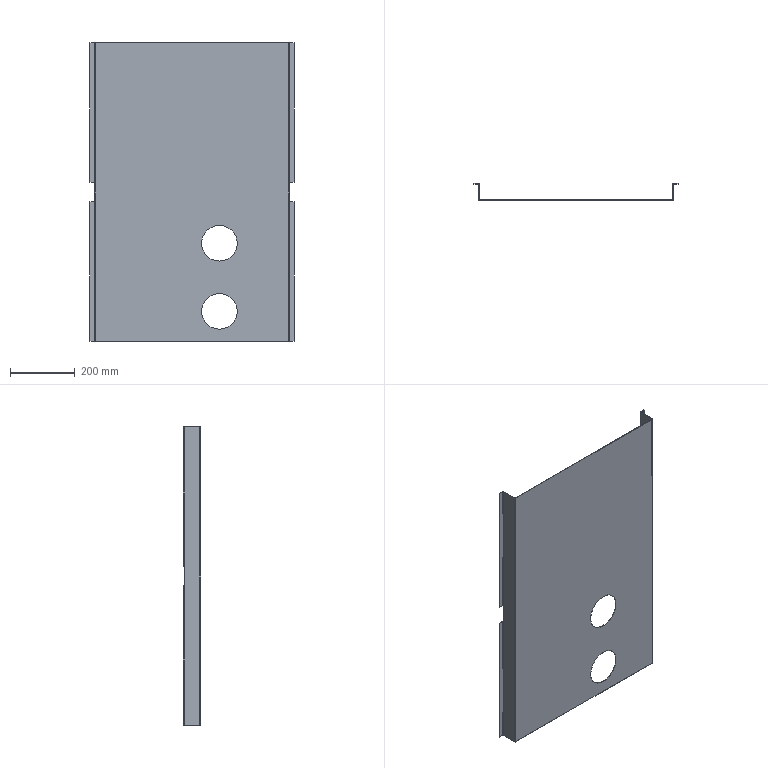Component | SolidWorks | LowerCrossbar400AType40001100-1 | 1 solid | 58 faces | volume 976520 mm3 | plane 42 | cylinder 16 | commonest cylinder face diameters 4.473 x6 1.473 x6 110 x4